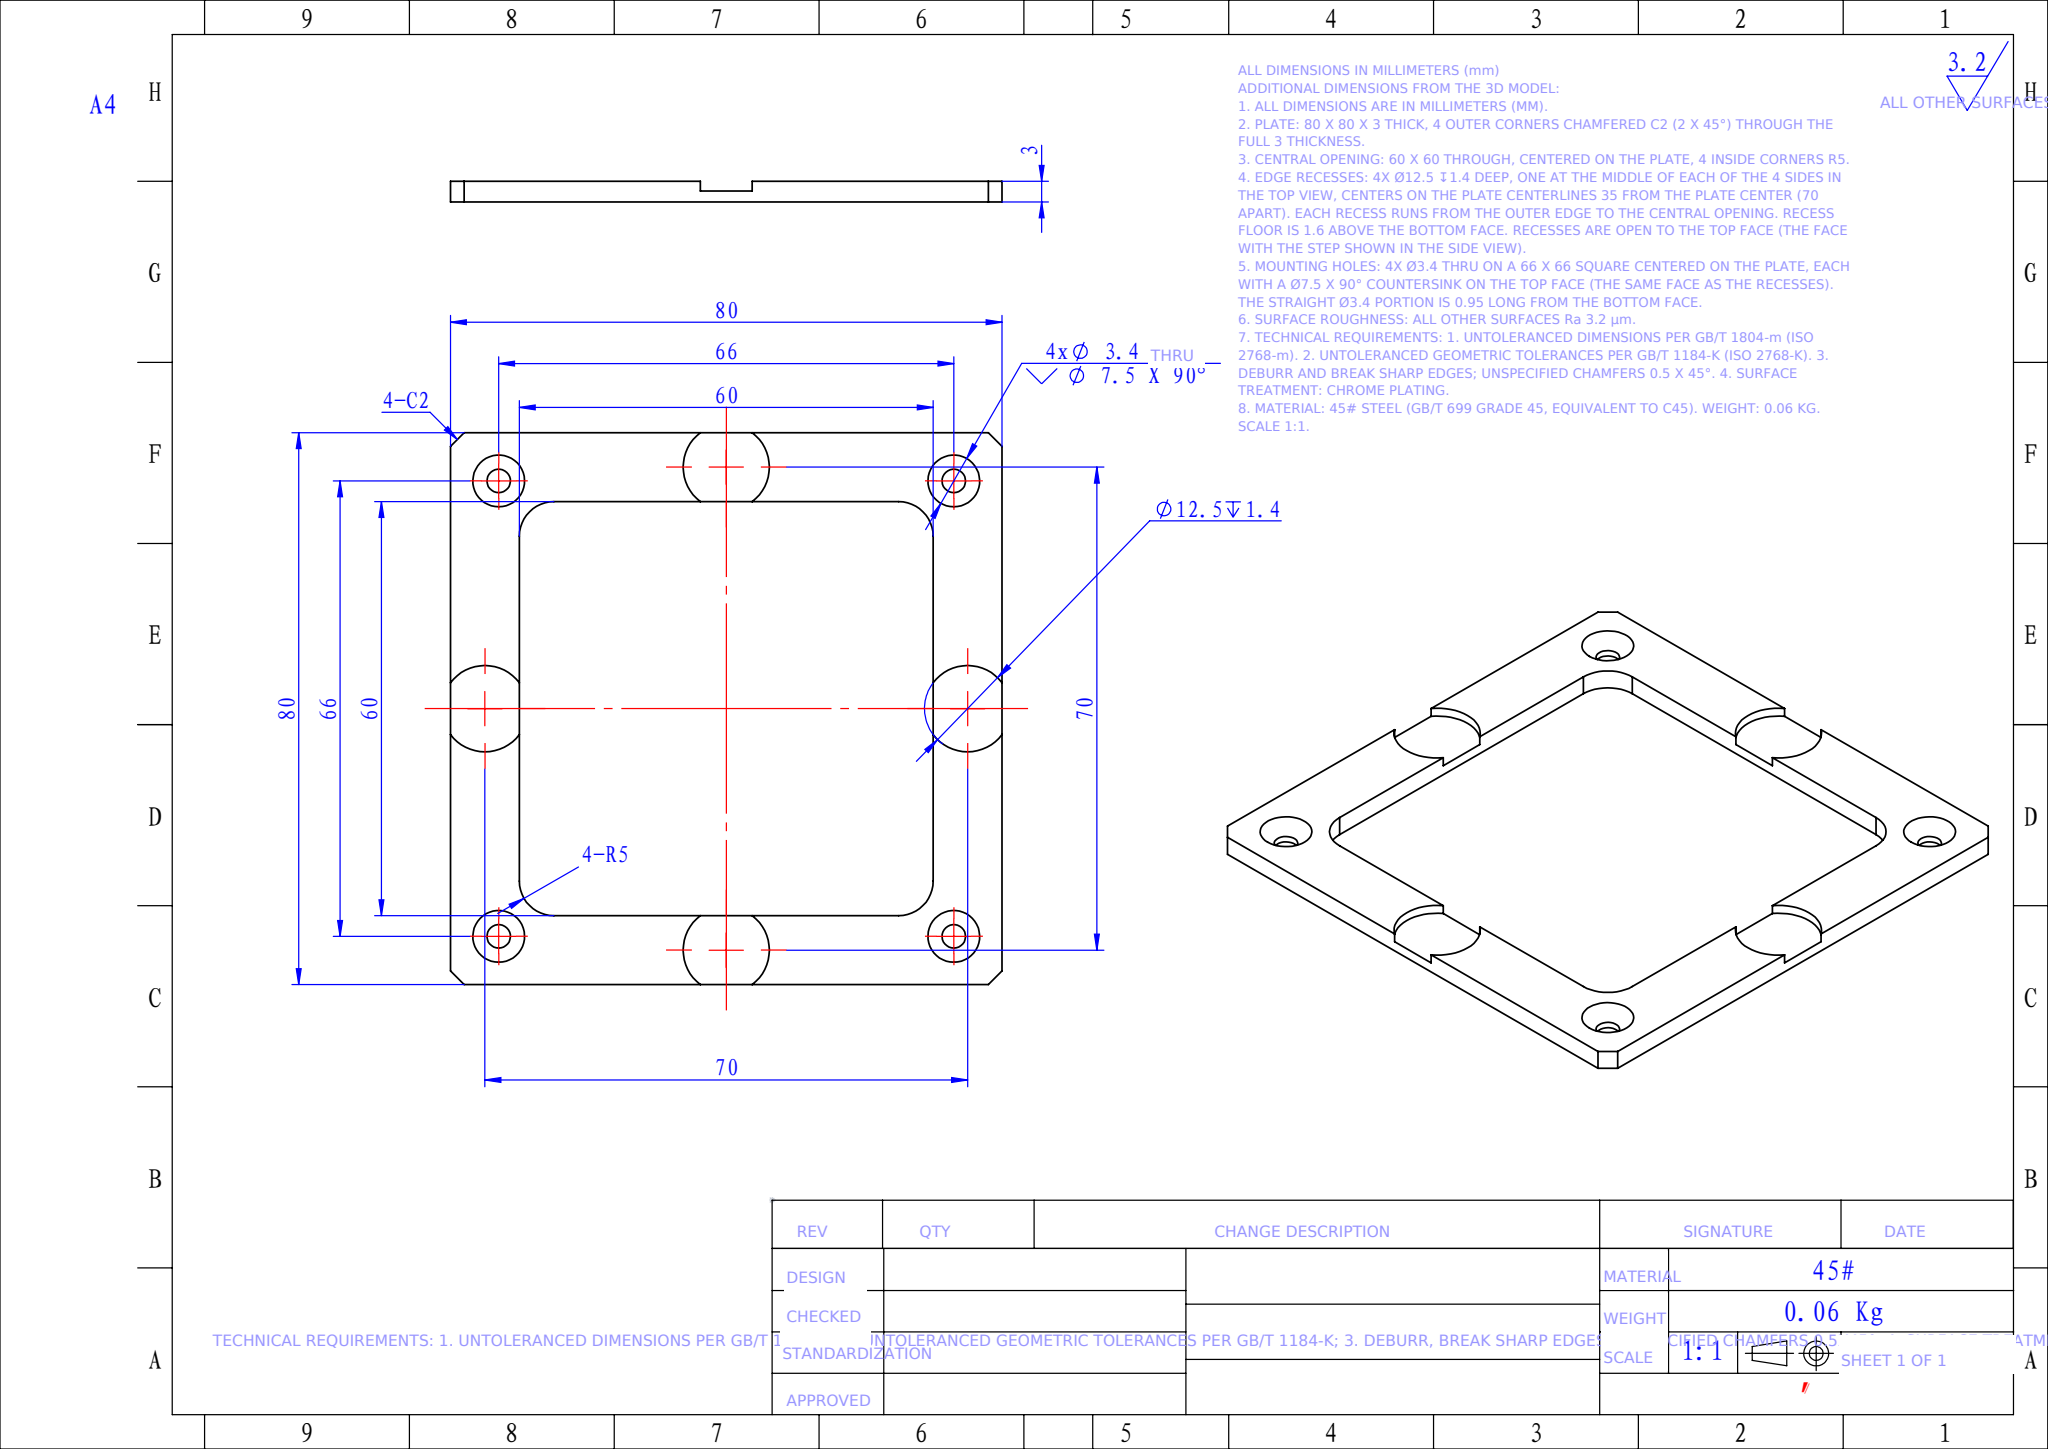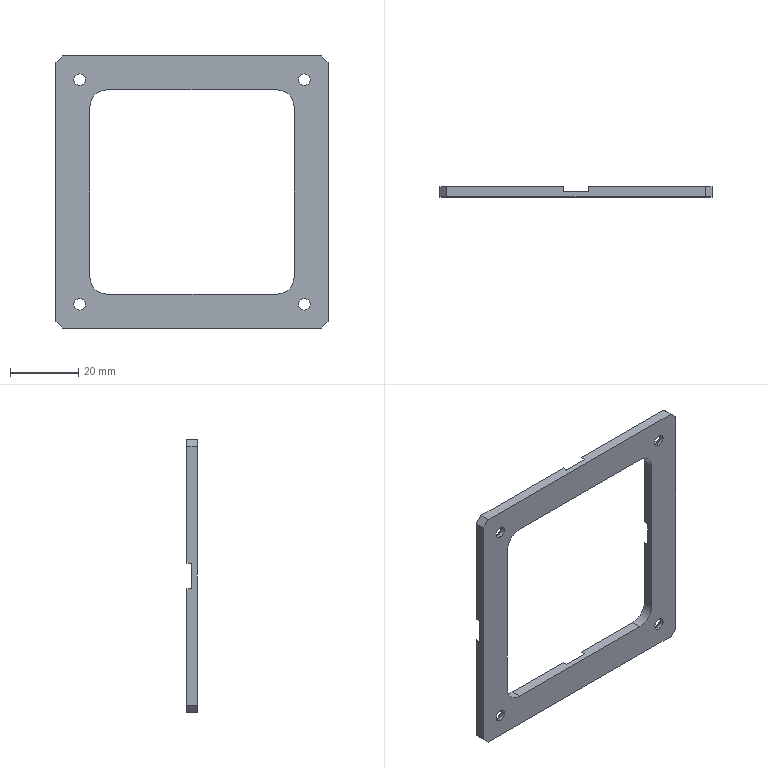Part | NX | mm | 1 solid | 51 faces | box 80 x 3 x 80 mm | volume 7590 mm3 | cylinder 22 | plane 21 | cone 8 | commonest cylinder face diameters 12.5 x10 3.4 x8 10 x4